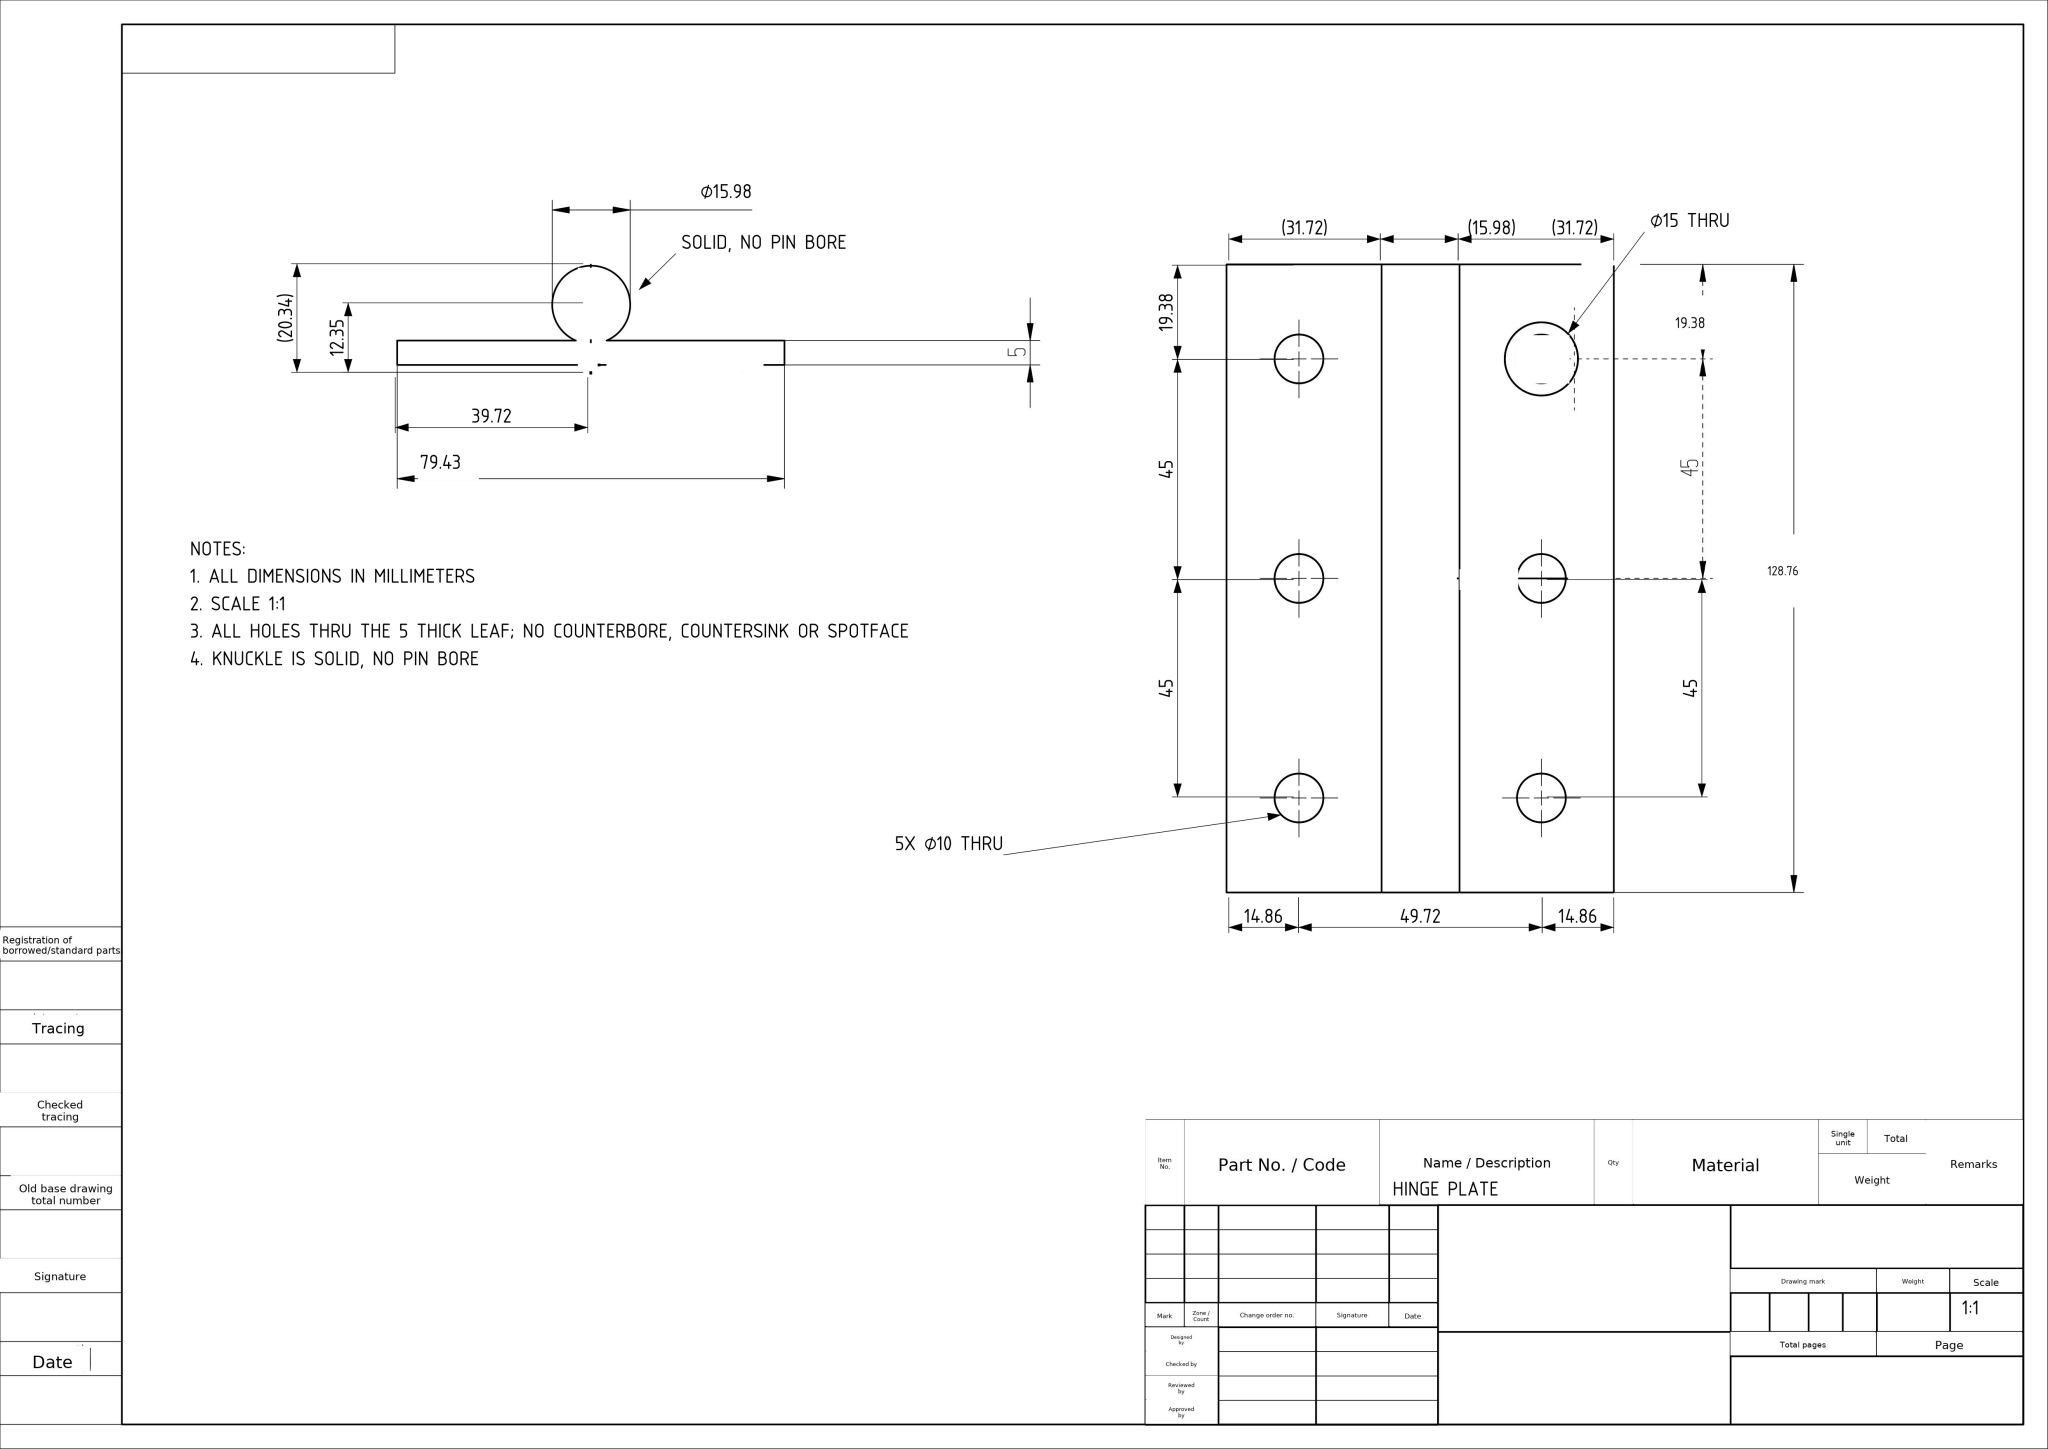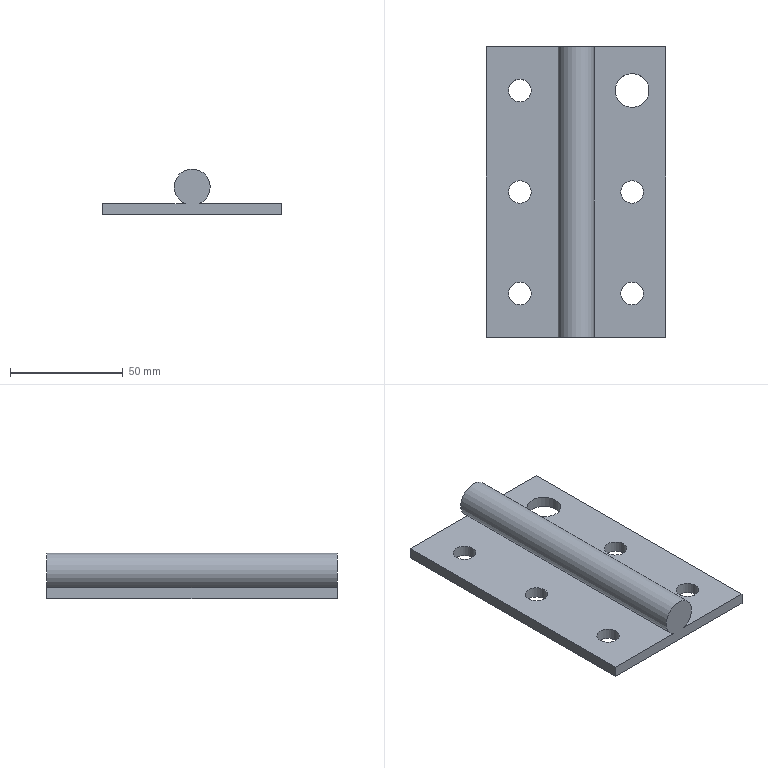Part | NX | mm | 1 solid | 14 faces | box 79.43 x 128.76 x 20.34 mm | volume 73777 mm3 | plane 7 | cylinder 7 | commonest cylinder face diameters 10 x5 15 x1 15.985 x1
STEP:
#1=CARTESIAN_POINT('',(0.,0.,0.));
#2=DIRECTION('',(0.,0.,1.));
#3=DIRECTION('',(1.,0.,0.));
#4=AXIS2_PLACEMENT_3D('',#1,#2,#3);
#5=(LENGTH_UNIT()NAMED_UNIT(*)SI_UNIT(.MILLI.,.METRE.));
#6=UNCERTAINTY_MEASURE_WITH_UNIT(LENGTH_MEASURE(0.00002),#5,'','');
#7=(NAMED_UNIT(*)PLANE_ANGLE_UNIT()SI_UNIT($,.RADIAN.));
#8=PLANE_ANGLE_MEASURE_WITH_UNIT(PLANE_ANGLE_MEASURE(0.01745),#7);
#9=DIMENSIONAL_EXPONENTS(0.,0.,0.,0.,0.,0.,0.);
#10=(CONVERSION_BASED_UNIT('',#8)NAMED_UNIT(#9)PLANE_ANGLE_UNIT());
#11=(NAMED_UNIT(*)SI_UNIT($,.STERADIAN.)SOLID_ANGLE_UNIT());
#12=(GEOMETRIC_REPRESENTATION_CONTEXT(3)GLOBAL_UNCERTAINTY_ASSIGNED_CONTEXT((#6))GLOBAL_UNIT_ASSIGNED_CONTEXT((#5,#10,#11))REPRESENTATION_CONTEXT('',''));
#13=SHAPE_REPRESENTATION('',(#4),#12);
#14=CARTESIAN_POINT('',(-29.86,45.,5.));
#15=VERTEX_POINT('',#14);
#16=CARTESIAN_POINT('',(-24.86,45.,5.));
#17=DIRECTION('',(0.,0.,-1.));
#18=DIRECTION('',(-1.,0.,0.));
#19=AXIS2_PLACEMENT_3D('',#16,#17,#18);
#20=CIRCLE('',#19,5.);
#21=EDGE_CURVE('',#15,#15,#20,.T.);
#22=ORIENTED_EDGE('',*,*,#21,.T.);
#23=EDGE_LOOP('',(#22));
#24=FACE_BOUND('',#23,.T.);
#25=CARTESIAN_POINT('',(-29.86,-45.,5.));
#26=VERTEX_POINT('',#25);
#27=CARTESIAN_POINT('',(-24.86,-45.,5.));
#28=DIRECTION('',(0.,0.,1.));
#29=DIRECTION('',(-1.,0.,0.));
#30=AXIS2_PLACEMENT_3D('',#27,#28,#29);
#31=CIRCLE('',#30,5.);
#32=EDGE_CURVE('',#26,#26,#31,.T.);
#33=ORIENTED_EDGE('',*,*,#32,.F.);
#34=EDGE_LOOP('',(#33));
#35=FACE_BOUND('',#34,.T.);
#36=CARTESIAN_POINT('',(-29.86,0.,5.));
#37=VERTEX_POINT('',#36);
#38=CARTESIAN_POINT('',(-24.86,0.,5.));
#39=DIRECTION('',(0.,0.,-1.));
#40=DIRECTION('',(-1.,0.,0.));
#41=AXIS2_PLACEMENT_3D('',#38,#39,#40);
#42=CIRCLE('',#41,5.);
#43=EDGE_CURVE('',#37,#37,#42,.T.);
#44=ORIENTED_EDGE('',*,*,#43,.T.);
#45=EDGE_LOOP('',(#44));
#46=FACE_BOUND('',#45,.T.);
#47=CARTESIAN_POINT('',(-3.072,64.378,5.));
#48=VERTEX_POINT('',#47);
#49=CARTESIAN_POINT('',(-3.072,-64.378,5.));
#50=VERTEX_POINT('',#49);
#51=CARTESIAN_POINT('',(-3.072,-95.,5.));
#52=DIRECTION('',(0.,-1.,0.));
#53=VECTOR('',#52,1.);
#54=LINE('',#51,#53);
#55=EDGE_CURVE('',#48,#50,#54,.T.);
#56=ORIENTED_EDGE('',*,*,#55,.F.);
#57=CARTESIAN_POINT('',(-39.716,64.378,5.));
#58=VERTEX_POINT('',#57);
#59=CARTESIAN_POINT('',(39.716,64.378,5.));
#60=DIRECTION('',(-1.,0.,0.));
#61=VECTOR('',#60,1.);
#62=LINE('',#59,#61);
#63=EDGE_CURVE('',#48,#58,#62,.T.);
#64=ORIENTED_EDGE('',*,*,#63,.T.);
#65=CARTESIAN_POINT('',(-39.716,-64.378,5.));
#66=VERTEX_POINT('',#65);
#67=CARTESIAN_POINT('',(-39.716,64.378,5.));
#68=DIRECTION('',(0.,-1.,0.));
#69=VECTOR('',#68,1.);
#70=LINE('',#67,#69);
#71=EDGE_CURVE('',#58,#66,#70,.T.);
#72=ORIENTED_EDGE('',*,*,#71,.T.);
#73=CARTESIAN_POINT('',(-39.716,-64.378,5.));
#74=DIRECTION('',(1.,0.,0.));
#75=VECTOR('',#74,1.);
#76=LINE('',#73,#75);
#77=EDGE_CURVE('',#66,#50,#76,.T.);
#78=ORIENTED_EDGE('',*,*,#77,.T.);
#79=EDGE_LOOP('',(#56,#64,#72,#78));
#80=FACE_BOUND('',#79,.T.);
#81=CARTESIAN_POINT('',(24.86,-45.,5.));
#82=DIRECTION('',(0.,0.,-1.));
#83=DIRECTION('',(-1.,0.,0.));
#84=AXIS2_PLACEMENT_3D('',#81,#82,#83);
#85=PLANE('',#84);
#86=ADVANCED_FACE('',(#24,#35,#46,#80),#85,.F.);
#87=CARTESIAN_POINT('',(29.86,0.,5.));
#88=VERTEX_POINT('',#87);
#89=CARTESIAN_POINT('',(24.86,0.,5.));
#90=DIRECTION('',(0.,0.,1.));
#91=DIRECTION('',(1.,0.,0.));
#92=AXIS2_PLACEMENT_3D('',#89,#90,#91);
#93=CIRCLE('',#92,5.);
#94=EDGE_CURVE('',#88,#88,#93,.T.);
#95=ORIENTED_EDGE('',*,*,#94,.F.);
#96=EDGE_LOOP('',(#95));
#97=FACE_BOUND('',#96,.T.);
#98=CARTESIAN_POINT('',(32.36,45.,5.));
#99=VERTEX_POINT('',#98);
#100=CARTESIAN_POINT('',(24.86,45.,5.));
#101=DIRECTION('',(0.,0.,1.));
#102=DIRECTION('',(1.,0.,0.));
#103=AXIS2_PLACEMENT_3D('',#100,#101,#102);
#104=CIRCLE('',#103,7.5);
#105=EDGE_CURVE('',#99,#99,#104,.T.);
#106=ORIENTED_EDGE('',*,*,#105,.F.);
#107=EDGE_LOOP('',(#106));
#108=FACE_BOUND('',#107,.T.);
#109=CARTESIAN_POINT('',(29.86,-45.,5.));
#110=VERTEX_POINT('',#109);
#111=CARTESIAN_POINT('',(24.86,-45.,5.));
#112=DIRECTION('',(0.,0.,-1.));
#113=DIRECTION('',(1.,0.,0.));
#114=AXIS2_PLACEMENT_3D('',#111,#112,#113);
#115=CIRCLE('',#114,5.);
#116=EDGE_CURVE('',#110,#110,#115,.T.);
#117=ORIENTED_EDGE('',*,*,#116,.T.);
#118=EDGE_LOOP('',(#117));
#119=FACE_BOUND('',#118,.T.);
#120=CARTESIAN_POINT('',(3.229,-64.378,5.));
#121=VERTEX_POINT('',#120);
#122=CARTESIAN_POINT('',(3.229,64.378,5.));
#123=VERTEX_POINT('',#122);
#124=CARTESIAN_POINT('',(3.229,-95.,5.));
#125=DIRECTION('',(0.,1.,0.));
#126=VECTOR('',#125,1.);
#127=LINE('',#124,#126);
#128=EDGE_CURVE('',#121,#123,#127,.T.);
#129=ORIENTED_EDGE('',*,*,#128,.F.);
#130=CARTESIAN_POINT('',(39.716,-64.378,5.));
#131=VERTEX_POINT('',#130);
#132=CARTESIAN_POINT('',(-39.716,-64.378,5.));
#133=DIRECTION('',(1.,0.,0.));
#134=VECTOR('',#133,1.);
#135=LINE('',#132,#134);
#136=EDGE_CURVE('',#121,#131,#135,.T.);
#137=ORIENTED_EDGE('',*,*,#136,.T.);
#138=CARTESIAN_POINT('',(39.716,64.378,5.));
#139=VERTEX_POINT('',#138);
#140=CARTESIAN_POINT('',(39.716,-64.378,5.));
#141=DIRECTION('',(0.,1.,0.));
#142=VECTOR('',#141,1.);
#143=LINE('',#140,#142);
#144=EDGE_CURVE('',#131,#139,#143,.T.);
#145=ORIENTED_EDGE('',*,*,#144,.T.);
#146=CARTESIAN_POINT('',(39.716,64.378,5.));
#147=DIRECTION('',(-1.,0.,0.));
#148=VECTOR('',#147,1.);
#149=LINE('',#146,#148);
#150=EDGE_CURVE('',#139,#123,#149,.T.);
#151=ORIENTED_EDGE('',*,*,#150,.T.);
#152=EDGE_LOOP('',(#129,#137,#145,#151));
#153=FACE_BOUND('',#152,.T.);
#154=CARTESIAN_POINT('',(24.86,-45.,5.));
#155=DIRECTION('',(0.,0.,-1.));
#156=DIRECTION('',(-1.,0.,0.));
#157=AXIS2_PLACEMENT_3D('',#154,#155,#156);
#158=PLANE('',#157);
#159=ADVANCED_FACE('',(#97,#108,#119,#153),#158,.F.);
#160=CARTESIAN_POINT('',(-39.716,64.378,0.));
#161=VERTEX_POINT('',#160);
#162=CARTESIAN_POINT('',(-39.716,-64.378,0.));
#163=VERTEX_POINT('',#162);
#164=CARTESIAN_POINT('',(-39.716,64.378,0.));
#165=DIRECTION('',(0.,-1.,0.));
#166=VECTOR('',#165,1.);
#167=LINE('',#164,#166);
#168=EDGE_CURVE('',#161,#163,#167,.T.);
#169=ORIENTED_EDGE('',*,*,#168,.T.);
#170=CARTESIAN_POINT('',(-39.716,-64.378,5.));
#171=DIRECTION('',(0.,0.,-1.));
#172=VECTOR('',#171,1.);
#173=LINE('',#170,#172);
#174=EDGE_CURVE('',#66,#163,#173,.T.);
#175=ORIENTED_EDGE('',*,*,#174,.F.);
#176=ORIENTED_EDGE('',*,*,#71,.F.);
#177=CARTESIAN_POINT('',(-39.716,64.378,5.));
#178=DIRECTION('',(0.,0.,-1.));
#179=VECTOR('',#178,1.);
#180=LINE('',#177,#179);
#181=EDGE_CURVE('',#58,#161,#180,.T.);
#182=ORIENTED_EDGE('',*,*,#181,.T.);
#183=EDGE_LOOP('',(#169,#175,#176,#182));
#184=FACE_OUTER_BOUND('',#183,.T.);
#185=CARTESIAN_POINT('',(-39.716,64.378,5.));
#186=DIRECTION('',(1.,0.,0.));
#187=DIRECTION('',(0.,0.,-1.));
#188=AXIS2_PLACEMENT_3D('',#185,#186,#187);
#189=PLANE('',#188);
#190=ADVANCED_FACE('',(#184),#189,.F.);
#191=ORIENTED_EDGE('',*,*,#136,.F.);
#192=CARTESIAN_POINT('',(0.07845,-64.378,12.345));
#193=DIRECTION('',(0.,1.,0.));
#194=DIRECTION('',(0.,0.,1.));
#195=AXIS2_PLACEMENT_3D('',#192,#193,#194);
#196=CIRCLE('',#195,7.992);
#197=EDGE_CURVE('',#50,#121,#196,.T.);
#198=ORIENTED_EDGE('',*,*,#197,.F.);
#199=ORIENTED_EDGE('',*,*,#77,.F.);
#200=ORIENTED_EDGE('',*,*,#174,.T.);
#201=CARTESIAN_POINT('',(39.716,-64.378,0.));
#202=VERTEX_POINT('',#201);
#203=CARTESIAN_POINT('',(-39.716,-64.378,0.));
#204=DIRECTION('',(1.,0.,0.));
#205=VECTOR('',#204,1.);
#206=LINE('',#203,#205);
#207=EDGE_CURVE('',#163,#202,#206,.T.);
#208=ORIENTED_EDGE('',*,*,#207,.T.);
#209=CARTESIAN_POINT('',(39.716,-64.378,5.));
#210=DIRECTION('',(0.,0.,-1.));
#211=VECTOR('',#210,1.);
#212=LINE('',#209,#211);
#213=EDGE_CURVE('',#131,#202,#212,.T.);
#214=ORIENTED_EDGE('',*,*,#213,.F.);
#215=EDGE_LOOP('',(#191,#198,#199,#200,#208,#214));
#216=FACE_OUTER_BOUND('',#215,.T.);
#217=CARTESIAN_POINT('',(-39.716,-64.378,5.));
#218=DIRECTION('',(0.,1.,0.));
#219=DIRECTION('',(0.,0.,1.));
#220=AXIS2_PLACEMENT_3D('',#217,#218,#219);
#221=PLANE('',#220);
#222=ADVANCED_FACE('',(#216),#221,.F.);
#223=CARTESIAN_POINT('',(39.716,64.378,0.));
#224=VERTEX_POINT('',#223);
#225=CARTESIAN_POINT('',(39.716,-64.378,0.));
#226=DIRECTION('',(0.,1.,0.));
#227=VECTOR('',#226,1.);
#228=LINE('',#225,#227);
#229=EDGE_CURVE('',#202,#224,#228,.T.);
#230=ORIENTED_EDGE('',*,*,#229,.T.);
#231=CARTESIAN_POINT('',(39.716,64.378,5.));
#232=DIRECTION('',(0.,0.,-1.));
#233=VECTOR('',#232,1.);
#234=LINE('',#231,#233);
#235=EDGE_CURVE('',#139,#224,#234,.T.);
#236=ORIENTED_EDGE('',*,*,#235,.F.);
#237=ORIENTED_EDGE('',*,*,#144,.F.);
#238=ORIENTED_EDGE('',*,*,#213,.T.);
#239=EDGE_LOOP('',(#230,#236,#237,#238));
#240=FACE_OUTER_BOUND('',#239,.T.);
#241=CARTESIAN_POINT('',(39.716,-64.378,5.));
#242=DIRECTION('',(-1.,0.,0.));
#243=DIRECTION('',(0.,0.,1.));
#244=AXIS2_PLACEMENT_3D('',#241,#242,#243);
#245=PLANE('',#244);
#246=ADVANCED_FACE('',(#240),#245,.F.);
#247=ORIENTED_EDGE('',*,*,#21,.F.);
#248=EDGE_LOOP('',(#247));
#249=FACE_BOUND('',#248,.T.);
#250=CARTESIAN_POINT('',(-29.86,45.,0.));
#251=VERTEX_POINT('',#250);
#252=CARTESIAN_POINT('',(-24.86,45.,0.));
#253=DIRECTION('',(0.,0.,-1.));
#254=DIRECTION('',(-1.,0.,0.));
#255=AXIS2_PLACEMENT_3D('',#252,#253,#254);
#256=CIRCLE('',#255,5.);
#257=EDGE_CURVE('',#251,#251,#256,.T.);
#258=ORIENTED_EDGE('',*,*,#257,.T.);
#259=EDGE_LOOP('',(#258));
#260=FACE_BOUND('',#259,.T.);
#261=CARTESIAN_POINT('',(-24.86,45.,5.));
#262=DIRECTION('',(0.,0.,-1.));
#263=DIRECTION('',(-1.,0.,0.));
#264=AXIS2_PLACEMENT_3D('',#261,#262,#263);
#265=CYLINDRICAL_SURFACE('',#264,5.);
#266=ADVANCED_FACE('',(#249,#260),#265,.F.);
#267=ORIENTED_EDGE('',*,*,#32,.T.);
#268=EDGE_LOOP('',(#267));
#269=FACE_BOUND('',#268,.T.);
#270=CARTESIAN_POINT('',(-29.86,-45.,0.));
#271=VERTEX_POINT('',#270);
#272=CARTESIAN_POINT('',(-24.86,-45.,0.));
#273=DIRECTION('',(0.,0.,1.));
#274=DIRECTION('',(-1.,0.,0.));
#275=AXIS2_PLACEMENT_3D('',#272,#273,#274);
#276=CIRCLE('',#275,5.);
#277=EDGE_CURVE('',#271,#271,#276,.T.);
#278=ORIENTED_EDGE('',*,*,#277,.F.);
#279=EDGE_LOOP('',(#278));
#280=FACE_BOUND('',#279,.T.);
#281=CARTESIAN_POINT('',(-24.86,-45.,5.));
#282=DIRECTION('',(0.,0.,-1.));
#283=DIRECTION('',(-1.,0.,0.));
#284=AXIS2_PLACEMENT_3D('',#281,#282,#283);
#285=CYLINDRICAL_SURFACE('',#284,5.);
#286=ADVANCED_FACE('',(#269,#280),#285,.F.);
#287=ORIENTED_EDGE('',*,*,#43,.F.);
#288=EDGE_LOOP('',(#287));
#289=FACE_BOUND('',#288,.T.);
#290=CARTESIAN_POINT('',(-29.86,0.,0.));
#291=VERTEX_POINT('',#290);
#292=CARTESIAN_POINT('',(-24.86,0.,0.));
#293=DIRECTION('',(0.,0.,-1.));
#294=DIRECTION('',(-1.,0.,0.));
#295=AXIS2_PLACEMENT_3D('',#292,#293,#294);
#296=CIRCLE('',#295,5.);
#297=EDGE_CURVE('',#291,#291,#296,.T.);
#298=ORIENTED_EDGE('',*,*,#297,.T.);
#299=EDGE_LOOP('',(#298));
#300=FACE_BOUND('',#299,.T.);
#301=CARTESIAN_POINT('',(-24.86,0.,5.));
#302=DIRECTION('',(0.,0.,-1.));
#303=DIRECTION('',(-1.,0.,0.));
#304=AXIS2_PLACEMENT_3D('',#301,#302,#303);
#305=CYLINDRICAL_SURFACE('',#304,5.);
#306=ADVANCED_FACE('',(#289,#300),#305,.F.);
#307=ORIENTED_EDGE('',*,*,#105,.T.);
#308=EDGE_LOOP('',(#307));
#309=FACE_BOUND('',#308,.T.);
#310=CARTESIAN_POINT('',(32.36,45.,0.));
#311=VERTEX_POINT('',#310);
#312=CARTESIAN_POINT('',(24.86,45.,0.));
#313=DIRECTION('',(0.,0.,1.));
#314=DIRECTION('',(1.,0.,0.));
#315=AXIS2_PLACEMENT_3D('',#312,#313,#314);
#316=CIRCLE('',#315,7.5);
#317=EDGE_CURVE('',#311,#311,#316,.T.);
#318=ORIENTED_EDGE('',*,*,#317,.F.);
#319=EDGE_LOOP('',(#318));
#320=FACE_BOUND('',#319,.T.);
#321=CARTESIAN_POINT('',(24.86,45.,5.));
#322=DIRECTION('',(0.,0.,-1.));
#323=DIRECTION('',(-1.,0.,0.));
#324=AXIS2_PLACEMENT_3D('',#321,#322,#323);
#325=CYLINDRICAL_SURFACE('',#324,7.5);
#326=ADVANCED_FACE('',(#309,#320),#325,.F.);
#327=ORIENTED_EDGE('',*,*,#116,.F.);
#328=EDGE_LOOP('',(#327));
#329=FACE_BOUND('',#328,.T.);
#330=CARTESIAN_POINT('',(29.86,-45.,0.));
#331=VERTEX_POINT('',#330);
#332=CARTESIAN_POINT('',(24.86,-45.,0.));
#333=DIRECTION('',(0.,0.,-1.));
#334=DIRECTION('',(1.,0.,0.));
#335=AXIS2_PLACEMENT_3D('',#332,#333,#334);
#336=CIRCLE('',#335,5.);
#337=EDGE_CURVE('',#331,#331,#336,.T.);
#338=ORIENTED_EDGE('',*,*,#337,.T.);
#339=EDGE_LOOP('',(#338));
#340=FACE_BOUND('',#339,.T.);
#341=CARTESIAN_POINT('',(24.86,-45.,5.));
#342=DIRECTION('',(0.,0.,-1.));
#343=DIRECTION('',(-1.,0.,0.));
#344=AXIS2_PLACEMENT_3D('',#341,#342,#343);
#345=CYLINDRICAL_SURFACE('',#344,5.);
#346=ADVANCED_FACE('',(#329,#340),#345,.F.);
#347=ORIENTED_EDGE('',*,*,#63,.F.);
#348=CARTESIAN_POINT('',(0.07845,64.378,12.345));
#349=DIRECTION('',(0.,-1.,0.));
#350=DIRECTION('',(0.,0.,-1.));
#351=AXIS2_PLACEMENT_3D('',#348,#349,#350);
#352=CIRCLE('',#351,7.992);
#353=EDGE_CURVE('',#123,#48,#352,.T.);
#354=ORIENTED_EDGE('',*,*,#353,.F.);
#355=ORIENTED_EDGE('',*,*,#150,.F.);
#356=ORIENTED_EDGE('',*,*,#235,.T.);
#357=CARTESIAN_POINT('',(39.716,64.378,0.));
#358=DIRECTION('',(-1.,0.,0.));
#359=VECTOR('',#358,1.);
#360=LINE('',#357,#359);
#361=EDGE_CURVE('',#224,#161,#360,.T.);
#362=ORIENTED_EDGE('',*,*,#361,.T.);
#363=ORIENTED_EDGE('',*,*,#181,.F.);
#364=EDGE_LOOP('',(#347,#354,#355,#356,#362,#363));
#365=FACE_OUTER_BOUND('',#364,.T.);
#366=CARTESIAN_POINT('',(39.716,64.378,5.));
#367=DIRECTION('',(0.,-1.,0.));
#368=DIRECTION('',(0.,0.,-1.));
#369=AXIS2_PLACEMENT_3D('',#366,#367,#368);
#370=PLANE('',#369);
#371=ADVANCED_FACE('',(#365),#370,.F.);
#372=ORIENTED_EDGE('',*,*,#94,.T.);
#373=EDGE_LOOP('',(#372));
#374=FACE_BOUND('',#373,.T.);
#375=CARTESIAN_POINT('',(29.86,0.,0.));
#376=VERTEX_POINT('',#375);
#377=CARTESIAN_POINT('',(24.86,0.,0.));
#378=DIRECTION('',(0.,0.,1.));
#379=DIRECTION('',(1.,0.,0.));
#380=AXIS2_PLACEMENT_3D('',#377,#378,#379);
#381=CIRCLE('',#380,5.);
#382=EDGE_CURVE('',#376,#376,#381,.T.);
#383=ORIENTED_EDGE('',*,*,#382,.F.);
#384=EDGE_LOOP('',(#383));
#385=FACE_BOUND('',#384,.T.);
#386=CARTESIAN_POINT('',(24.86,0.,5.));
#387=DIRECTION('',(0.,0.,-1.));
#388=DIRECTION('',(-1.,0.,0.));
#389=AXIS2_PLACEMENT_3D('',#386,#387,#388);
#390=CYLINDRICAL_SURFACE('',#389,5.);
#391=ADVANCED_FACE('',(#374,#385),#390,.F.);
#392=ORIENTED_EDGE('',*,*,#168,.F.);
#393=ORIENTED_EDGE('',*,*,#361,.F.);
#394=ORIENTED_EDGE('',*,*,#229,.F.);
#395=ORIENTED_EDGE('',*,*,#207,.F.);
#396=EDGE_LOOP('',(#392,#393,#394,#395));
#397=FACE_BOUND('',#396,.T.);
#398=ORIENTED_EDGE('',*,*,#337,.F.);
#399=EDGE_LOOP('',(#398));
#400=FACE_BOUND('',#399,.T.);
#401=ORIENTED_EDGE('',*,*,#317,.T.);
#402=EDGE_LOOP('',(#401));
#403=FACE_BOUND('',#402,.T.);
#404=ORIENTED_EDGE('',*,*,#297,.F.);
#405=EDGE_LOOP('',(#404));
#406=FACE_BOUND('',#405,.T.);
#407=ORIENTED_EDGE('',*,*,#277,.T.);
#408=EDGE_LOOP('',(#407));
#409=FACE_BOUND('',#408,.T.);
#410=ORIENTED_EDGE('',*,*,#257,.F.);
#411=EDGE_LOOP('',(#410));
#412=FACE_BOUND('',#411,.T.);
#413=ORIENTED_EDGE('',*,*,#382,.T.);
#414=EDGE_LOOP('',(#413));
#415=FACE_BOUND('',#414,.T.);
#416=CARTESIAN_POINT('',(24.86,-45.,0.));
#417=DIRECTION('',(0.,0.,-1.));
#418=DIRECTION('',(-1.,0.,0.));
#419=AXIS2_PLACEMENT_3D('',#416,#417,#418);
#420=PLANE('',#419);
#421=ADVANCED_FACE('',(#397,#400,#403,#406,#409,#412,#415),#420,.T.);
#422=ORIENTED_EDGE('',*,*,#197,.T.);
#423=ORIENTED_EDGE('',*,*,#128,.T.);
#424=ORIENTED_EDGE('',*,*,#353,.T.);
#425=ORIENTED_EDGE('',*,*,#55,.T.);
#426=EDGE_LOOP('',(#422,#423,#424,#425));
#427=FACE_OUTER_BOUND('',#426,.T.);
#428=CARTESIAN_POINT('',(0.07845,-95.,12.345));
#429=DIRECTION('',(0.,1.,0.));
#430=DIRECTION('',(0.,0.,1.));
#431=AXIS2_PLACEMENT_3D('',#428,#429,#430);
#432=CYLINDRICAL_SURFACE('',#431,7.992);
#433=ADVANCED_FACE('',(#427),#432,.T.);
#434=CLOSED_SHELL('',(#86,#159,#190,#222,#246,#266,#286,#306,#326,#346,#371,#391,#421,#433));
#435=MANIFOLD_SOLID_BREP('',#434);
#436=ADVANCED_BREP_SHAPE_REPRESENTATION('',(#435),#12);
#437=SHAPE_REPRESENTATION_RELATIONSHIP('','',#13,#436);
#438=PRESENTATION_LAYER_ASSIGNMENT('','',(#435));
#439=COLOUR_RGB('',1.,0.6,0.);
#440=FILL_AREA_STYLE_COLOUR('',#439);
#441=FILL_AREA_STYLE('',(#440));
#442=SURFACE_STYLE_FILL_AREA(#441);
#443=SURFACE_SIDE_STYLE('',(#442));
#444=SURFACE_STYLE_USAGE(.BOTH.,#443);
#445=PRESENTATION_STYLE_ASSIGNMENT((#444));
#446=STYLED_ITEM('',(#445),#435);
#447=MECHANICAL_DESIGN_GEOMETRIC_PRESENTATION_REPRESENTATION('',(#446),#12);